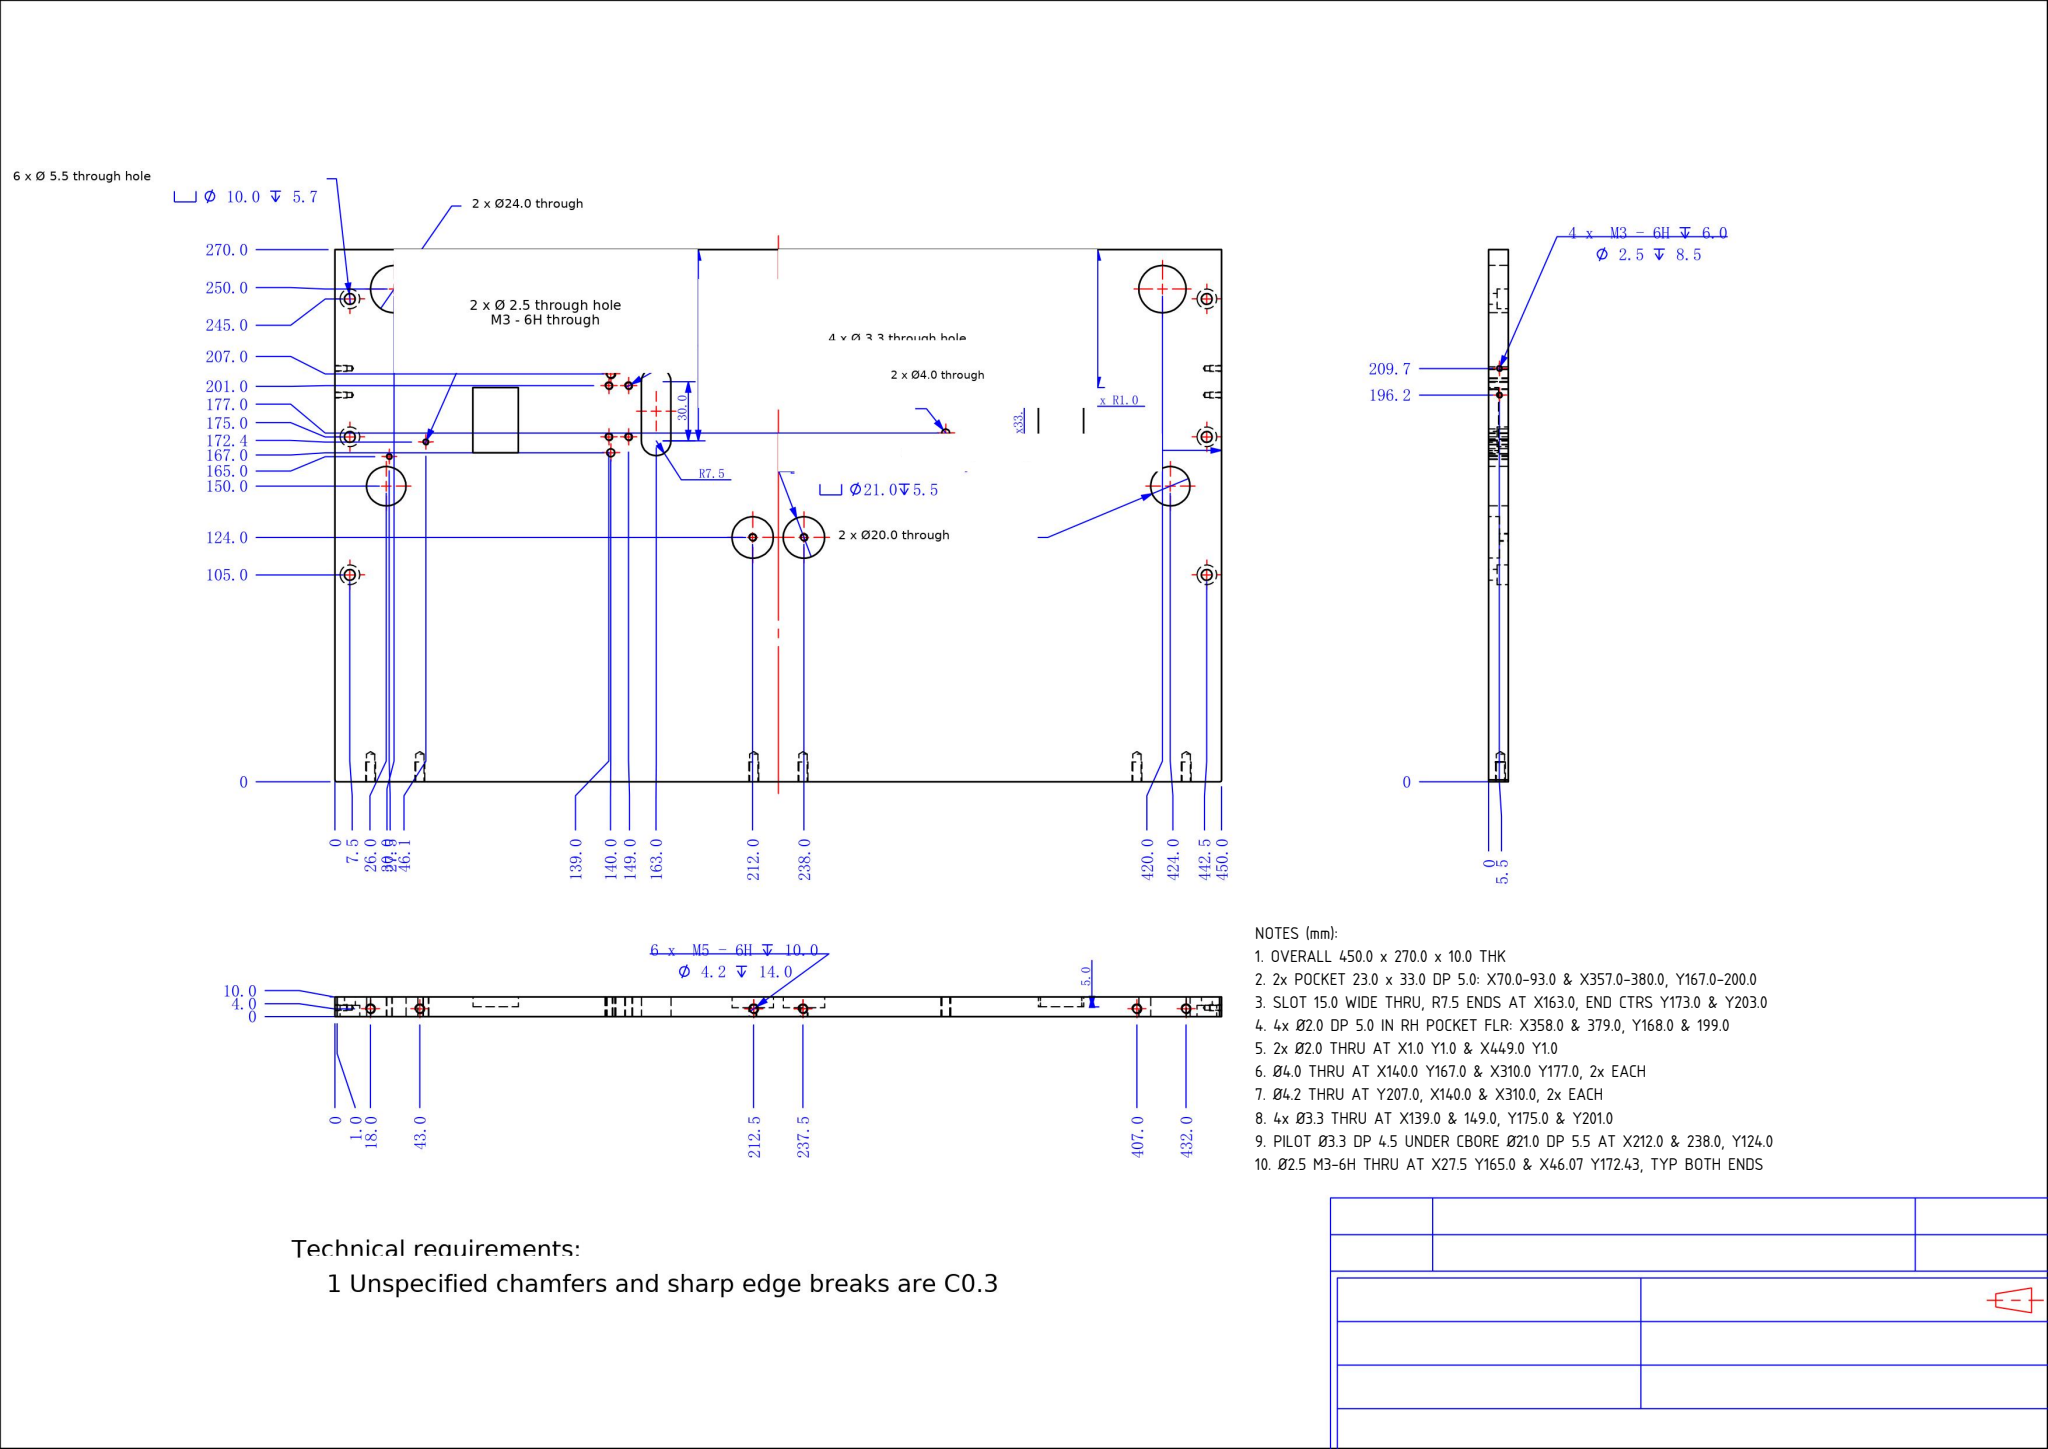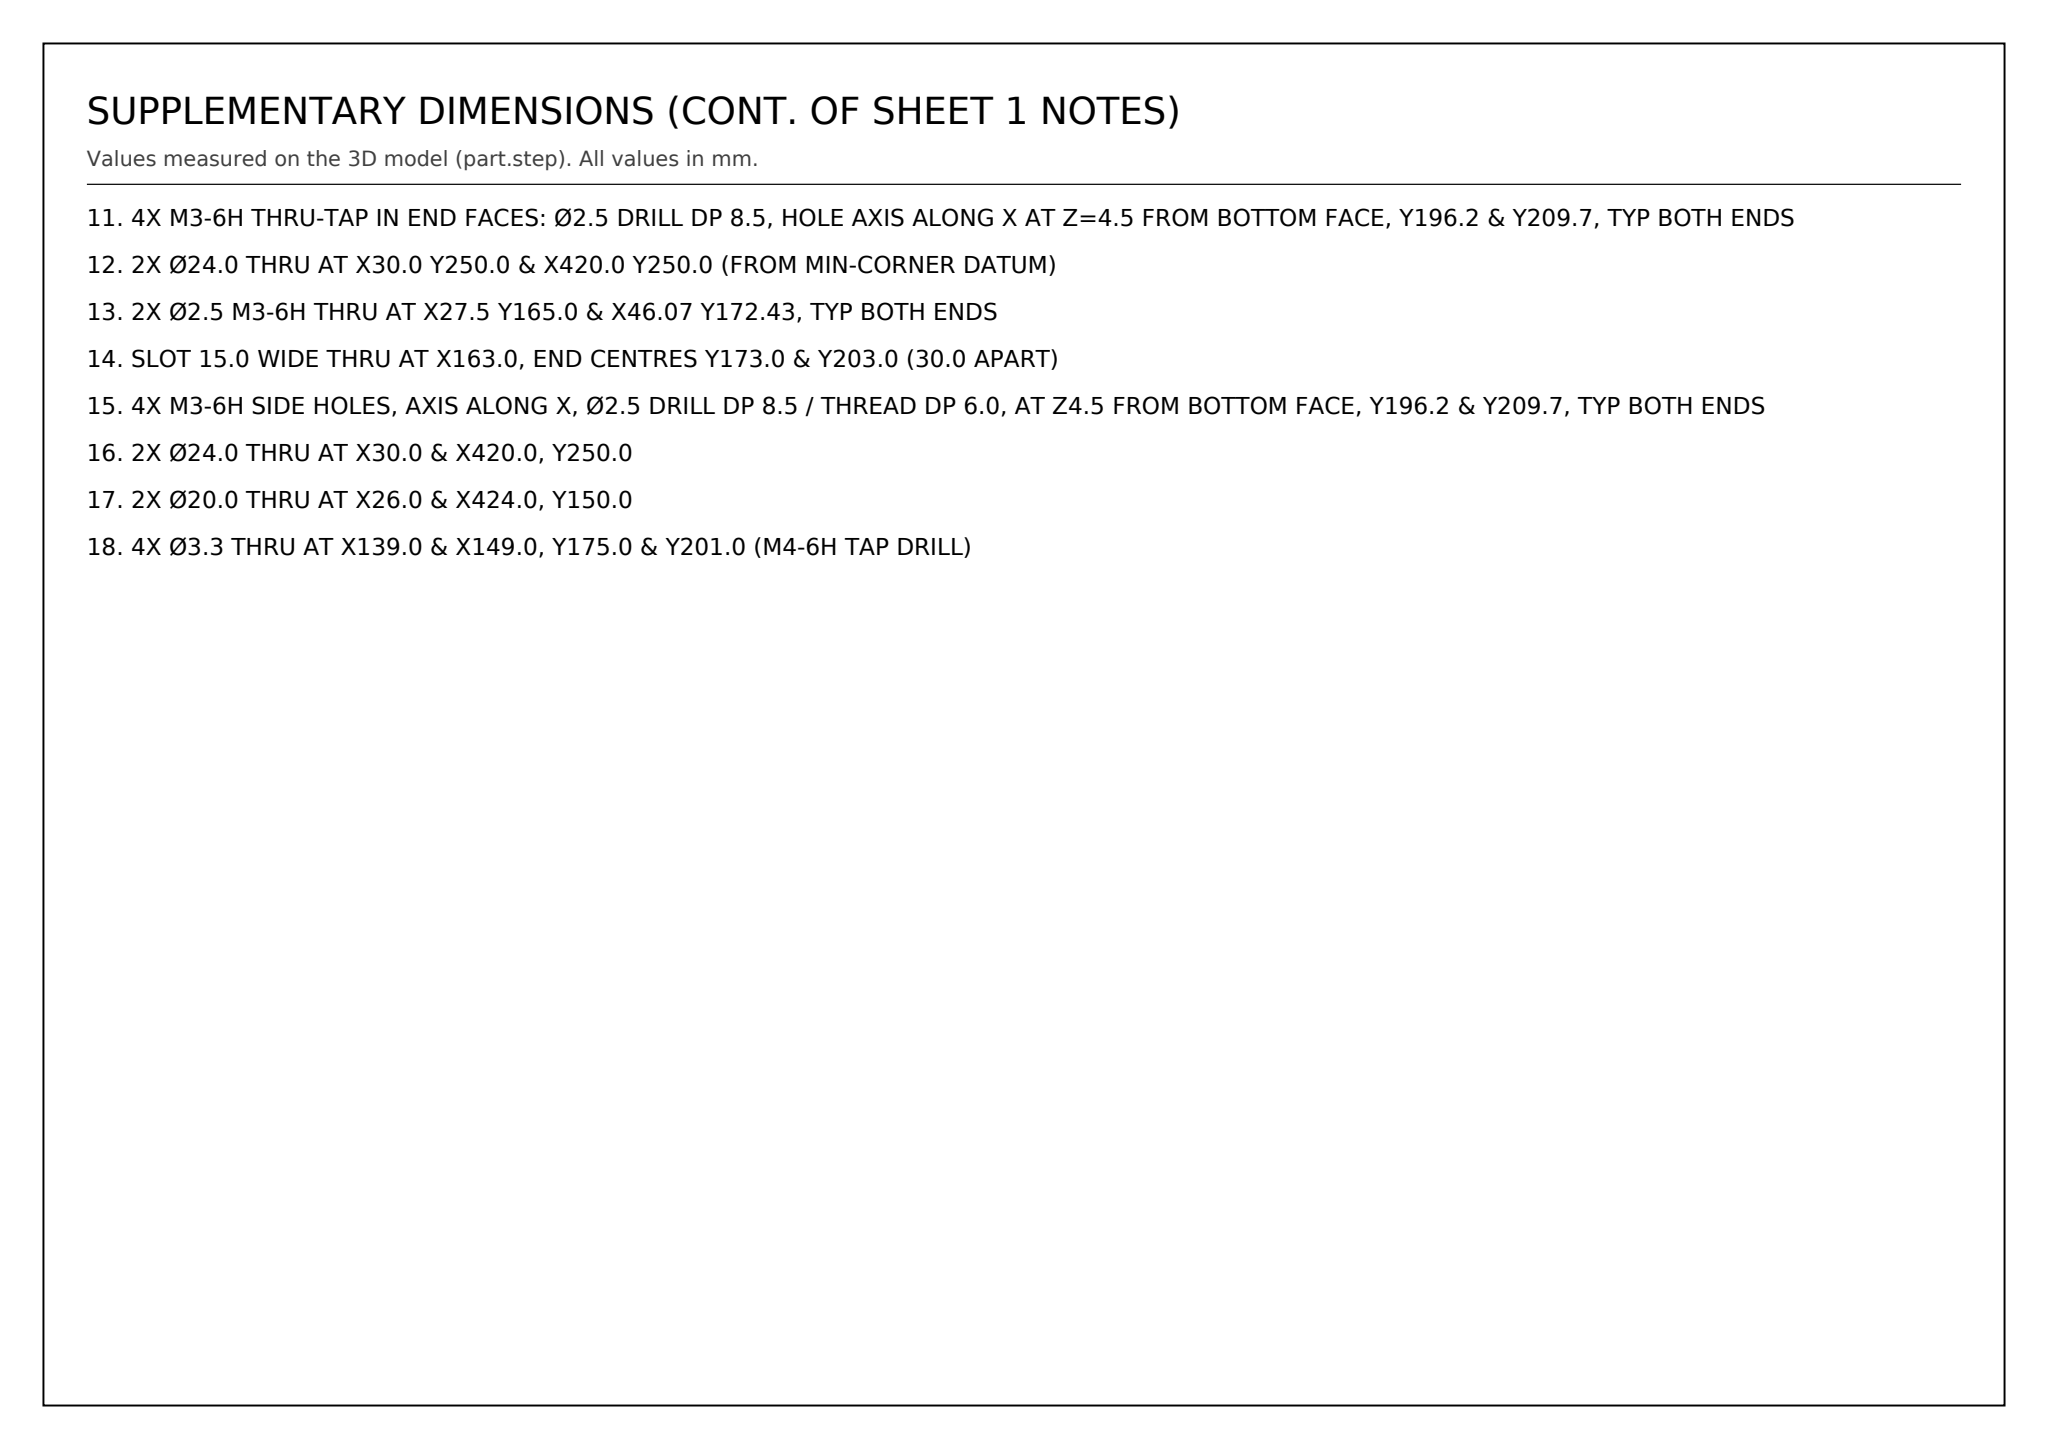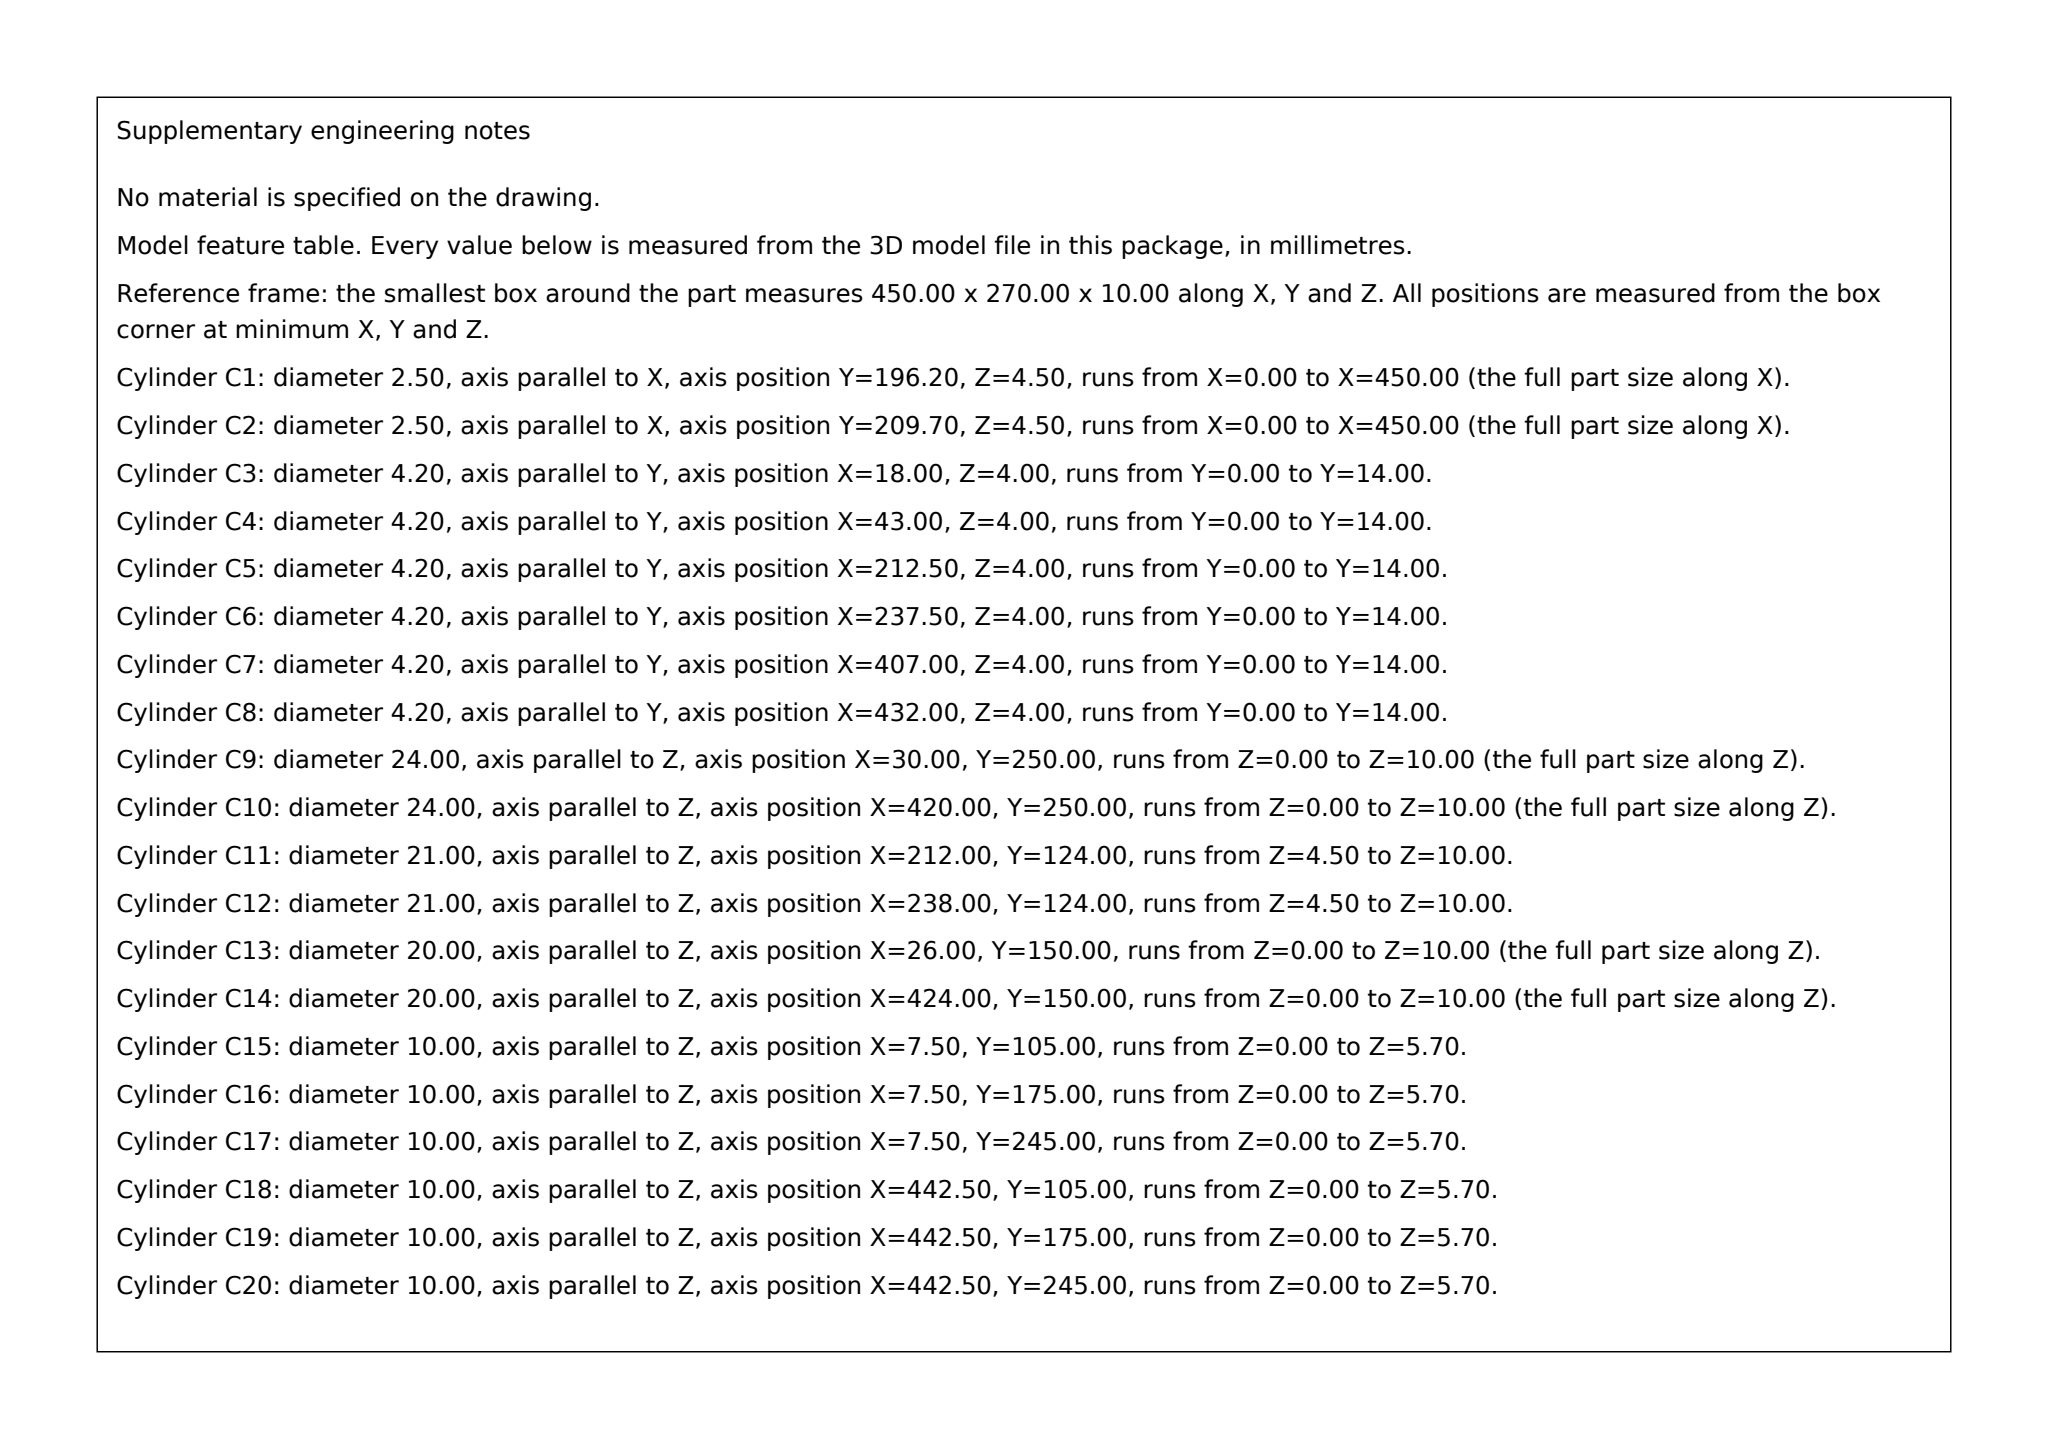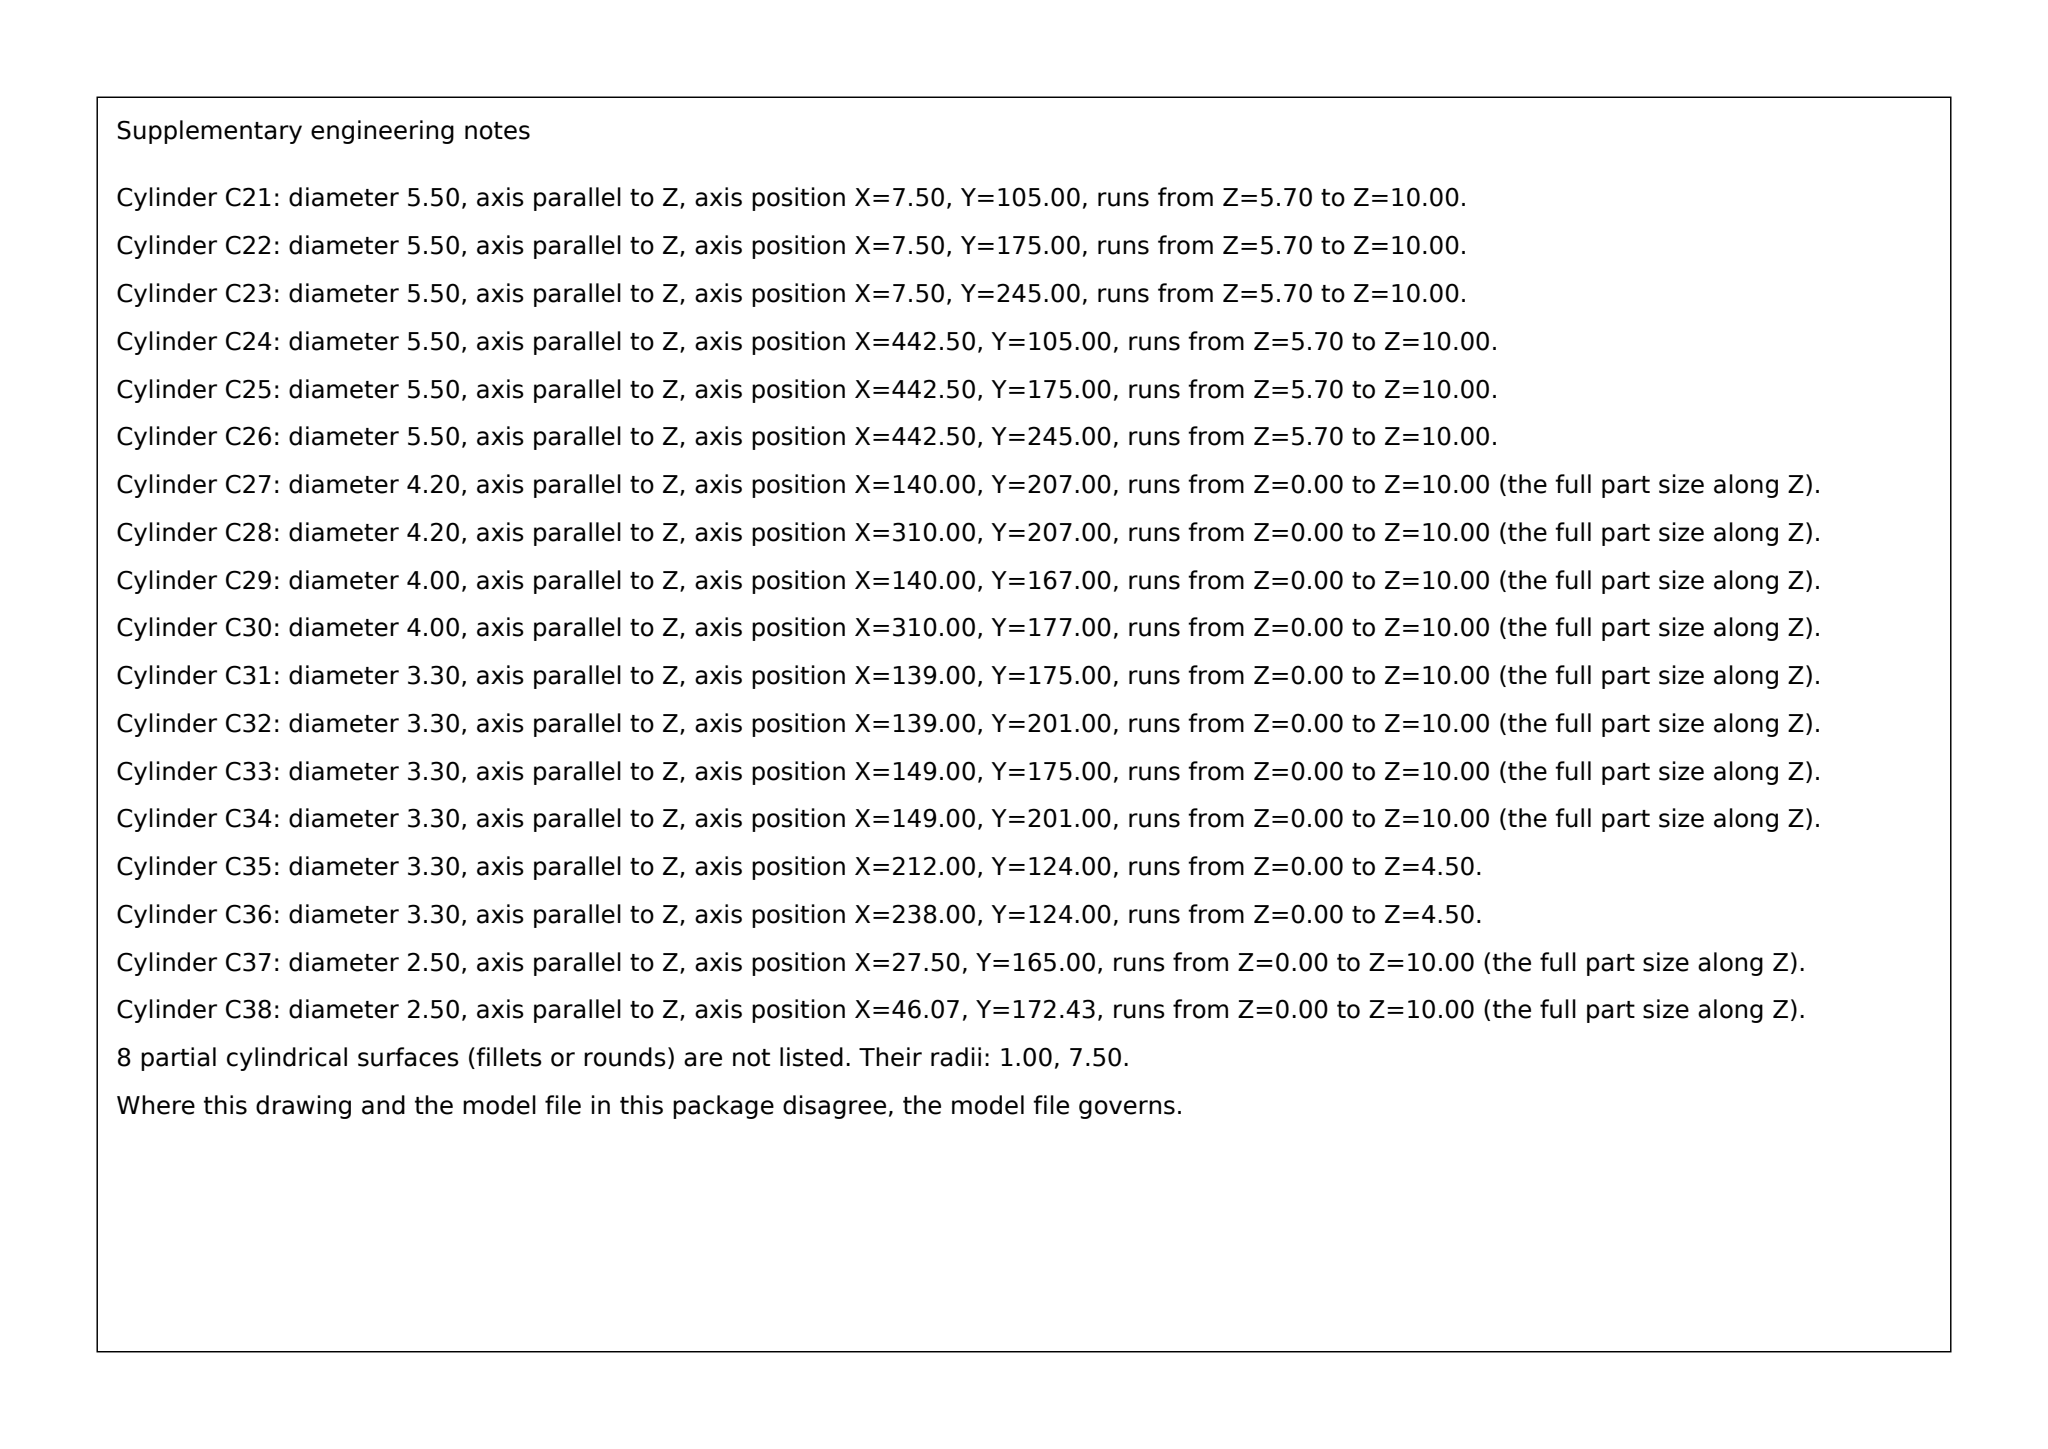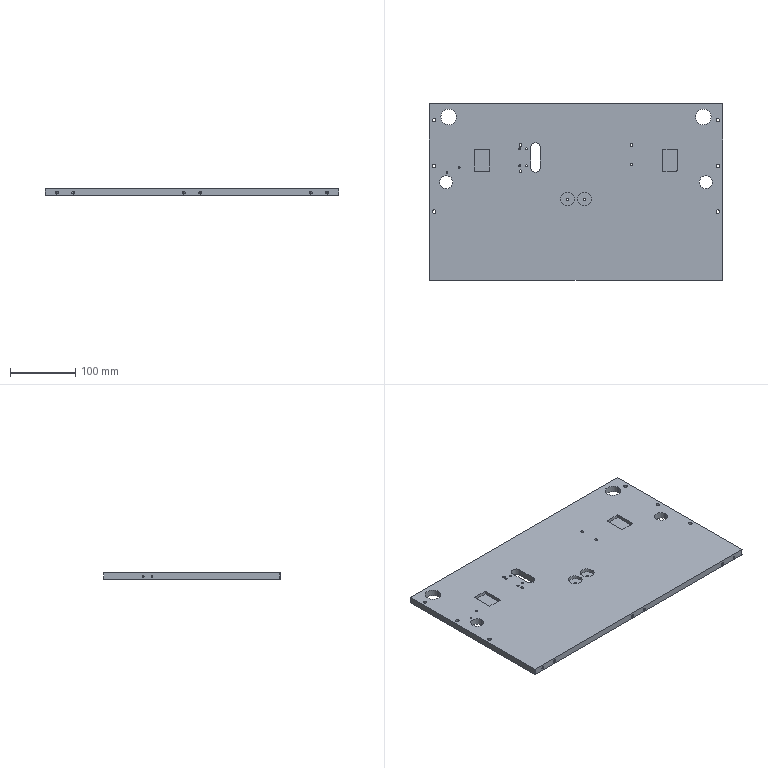Part | SolidWorks | mm | 1 solid | 134 faces | box 450 x 270 x 10 mm | volume 1176287 mm3 | cylinder 88 | plane 26 | cone 20 | commonest cylinder face diameters 4.2 x16 3.3 x12 2.5 x12 10 x12 5.5 x12 2 x6 21 x4 4 x4
Drawing notes:
OVERALL 450.0 x 270.0 x 10.0 THK | from the solid: bbox_xyz 450.0 x 270.0 x 10.0
2x POCKET 23.0 x 33.0 DP 5.0: X70.0-93.0 & X357.0-380.0, Y167.0-200.0 | from the solid: axis_planes x=70/93 & x=357/380, y=167(2) & y=200(2), z=5.0(2)
SLOT 15.0 WIDE THRU, R7.5 ENDS AT X163.0, END CTRS Y173.0 & Y203.0 | from the solid: Ø15.0 z-cyls at (163.0,173.0) & (163.0,203.0) len 10.0; walls x=155.5 & 170.5
4x Ø2.0 DP 5.0 IN RH POCKET FLR: X358.0 & 379.0, Y168.0 & 199.0 | from the solid: 4x Ø2.0 z-axis len 5.0 at (358/379, 168/199); pocket DP 5.0
2x Ø2.0 THRU AT X1.0 Y1.0 & X449.0 Y1.0 | from the solid: cylinders Ø2.0 z-axis at (1.0,1.0) & (449.0,1.0), length 10.0 = full thk
Ø4.0 THRU AT X140.0 Y167.0 & X310.0 Y177.0, 2x EACH | from the solid: 4.0 z @(140,167) len10 cnt2; 4.0 z @(310,177) len10 cnt2
Ø4.2 THRU AT Y207.0, X140.0 & X310.0, 2x EACH | from the solid: 4.2 z @(140,207) & (310,207) len 10 cnt2
4x Ø3.3 THRU AT X139.0 & 149.0, Y175.0 & Y201.0 | from the solid: 3.3 z @(139/149, 175/201) len 10
PILOT Ø3.3 DP 4.5 UNDER CBORE Ø21.0 DP 5.5 AT X212.0 & 238.0, Y124.0 | from the solid: 21.0 z @(212/238,124) len5.5; 3.3 z same pos len4.5
Ø2.5 M3-6H THRU AT X27.5 Y165.0 & X46.07 Y172.43, TYP BOTH ENDS | from the solid: 2.5 z @(27.5,165.0) & (46.07,172.43) len 10, cnt 2 each
4X M3-6H THRU-TAP IN END FACES: Ø2.5 DRILL DP 8.5, HOLE AXIS ALONG X AT Z=4.5 FROM BOTTOM FACE, Y196.2 & Y209.7, TYP BOTH ENDS | from the solid: cylinders dia 2.5, axis x, pos [-,196.2,4.5] and [-,209.7,4.5], length 8.5
2X Ø24.0 THRU AT X30.0 Y250.0 & X420.0 Y250.0 (FROM MIN-CORNER DATUM) | from the solid: cylinders dia 24.0, axis z, pos [30.0,250.0] and [420.0,250.0], length 10.0 (full 10.0 thk)
2X Ø2.5 M3-6H THRU AT X27.5 Y165.0 & X46.07 Y172.43, TYP BOTH ENDS | from the solid: cylinders dia 2.5, axis z, pos [27.5,165.0] and [46.07,172.43], length 10.0, count 2 each
SLOT 15.0 WIDE THRU AT X163.0, END CENTRES Y173.0 & Y203.0 (30.0 APART) | from the solid: cylinders dia 15.0, axis z, pos [163.0,173.0] and [163.0,203.0], length 10.0; planes x155.5 and x170.5
4X M3-6H SIDE HOLES, AXIS ALONG X, Ø2.5 DRILL DP 8.5 / THREAD DP 6.0, AT Z4.5 FROM BOTTOM FACE, Y196.2 & Y209.7, TYP BOTH ENDS | from the solid: cylinders dia 2.5 axis x at [y196.2, z4.5] len 8.5 (x4) and [y209.7, z4.5] len 8.5 (x4)
2X Ø24.0 THRU AT X30.0 & X420.0, Y250.0 | from the solid: cylinders dia 24.0 axis z at (30.0,250.0) and (420.0,250.0), length 10.0 = full 10.0 thk
2X Ø20.0 THRU AT X26.0 & X424.0, Y150.0 | from the solid: cylinders dia 20.0 axis z at (26.0,150.0) and (424.0,150.0), length 10.0 = full 10.0 thk
4X Ø3.3 THRU AT X139.0 & X149.0, Y175.0 & Y201.0 (M4-6H TAP DRILL) | from the solid: cylinders dia 3.3 axis z at (139/149, 175/201), length 10.0 full thickness